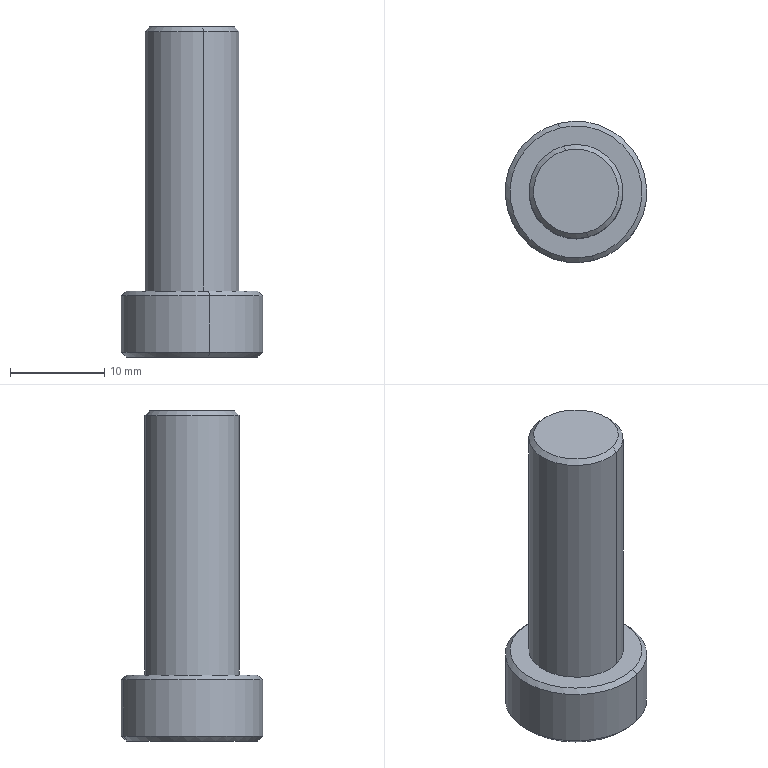Component | SolidWorks | JYTBJ-HeaderPlateBrakeAxis-1 | 1 solid | 17 faces | box 15 x 15 x 35 mm | volume 3077 mm3 | cone 8 | cylinder 6 | plane 3 | commonest cylinder face diameters 5 x2 10 x2 15 x2
build123d program:
from build123d import *

# Parameters (mm, degrees)
M6_TAPPED_HOLE1_D     = 5
M6_TAPPED_HOLE1_DEPTH = 17
M6_TAPPED_HOLE1_TIP   = 1.502
CHAMFER1_SIZE         = 0.5


with BuildPart() as part:
    # Sketch1 → Revolve1 (revolve)
    with BuildSketch(Plane.XY, mode=Mode.PRIVATE) as revolve1_sk:
        Polygon((0, 0), (7.5, 0), (7.5, 7), (5, 7), (5, 35), (0, 35), align=None)
    revolve(revolve1_sk.sketch.rotate(Axis((0, 0, 0), (0, 1, 0)), 90), axis=Axis((0, 0, 0), (0, 1, 0)))

    # M6 Tapped Hole1
    with Locations(Plane.XZ):
        with Locations((0, 0)):
            Hole(M6_TAPPED_HOLE1_D / 2, depth=M6_TAPPED_HOLE1_DEPTH)
            with Locations((0, 0, -(M6_TAPPED_HOLE1_DEPTH + M6_TAPPED_HOLE1_TIP / 2))):  # 118° drill point
                Cone(0, M6_TAPPED_HOLE1_D / 2, M6_TAPPED_HOLE1_TIP, mode=Mode.SUBTRACT)

    # Chamfer1
    chamfer1_edges = [part.edges().sort_by_distance(p)[0] for p in [
        (0, 35, 5),
        (0, 7, 7.5),
        (0, 0, 7.5),
    ]]
    chamfer(chamfer1_edges, length=CHAMFER1_SIZE)


solid = part.part

# Placed as in the assembly
solid = solid.moved(Location((35.724, 265.147, 18), (90, 0, 0)))
STEP:
#1=CARTESIAN_POINT('',(1.338,10.706,0.7087));
#2=VERTEX_POINT('',#1);
#3=CARTESIAN_POINT('',(1.475,10.172,0.7087));
#4=VERTEX_POINT('',#3);
#5=CARTESIAN_POINT('',(1.406,10.439,0.7087));
#6=DIRECTION('',(0.,0.,-1.));
#7=DIRECTION('',(-0.2502,0.9682,0.));
#8=AXIS2_PLACEMENT_3D('',#5,#6,#7);
#9=CIRCLE('',#8,0.2756);
#10=EDGE_CURVE('',#2,#4,#9,.T.);
#11=ORIENTED_EDGE('',*,*,#10,.F.);
#12=CARTESIAN_POINT('',(1.333,10.725,0.7283));
#13=VERTEX_POINT('',#12);
#14=CARTESIAN_POINT('',(1.338,10.706,0.7087));
#15=DIRECTION('',(-0.1769,0.6846,0.7071));
#16=VECTOR('',#15,39.37);
#17=LINE('',#14,#16);
#18=EDGE_CURVE('',#2,#13,#17,.T.);
#19=ORIENTED_EDGE('',*,*,#18,.T.);
#20=CARTESIAN_POINT('',(1.48,10.153,0.7283));
#21=VERTEX_POINT('',#20);
#22=CARTESIAN_POINT('',(1.406,10.439,0.7283));
#23=DIRECTION('',(0.,0.,1.));
#24=DIRECTION('',(-0.2502,0.9682,0.));
#25=AXIS2_PLACEMENT_3D('',#22,#23,#24);
#26=CIRCLE('',#25,0.2953);
#27=EDGE_CURVE('',#21,#13,#26,.T.);
#28=ORIENTED_EDGE('',*,*,#27,.F.);
#29=CARTESIAN_POINT('',(1.475,10.172,0.7087));
#30=DIRECTION('',(0.1769,-0.6846,0.7071));
#31=VECTOR('',#30,39.37);
#32=LINE('',#29,#31);
#33=EDGE_CURVE('',#4,#21,#32,.T.);
#34=ORIENTED_EDGE('',*,*,#33,.F.);
#35=EDGE_LOOP('',(#11,#19,#28,#34));
#36=FACE_OUTER_BOUND('',#35,.T.);
#37=CARTESIAN_POINT('',(1.406,10.439,0.7087));
#38=DIRECTION('',(0.,0.,1.));
#39=DIRECTION('',(0.2502,-0.9682,0.));
#40=AXIS2_PLACEMENT_3D('',#37,#38,#39);
#41=CONICAL_SURFACE('',#40,0.2756,0.7854);
#42=ADVANCED_FACE('',(#36),#41,.T.);
#43=CARTESIAN_POINT('',(1.475,10.172,0.9843));
#44=VERTEX_POINT('',#43);
#45=CARTESIAN_POINT('',(1.338,10.706,0.9843));
#46=VERTEX_POINT('',#45);
#47=CARTESIAN_POINT('',(1.406,10.439,0.9843));
#48=DIRECTION('',(0.,0.,1.));
#49=DIRECTION('',(0.2502,-0.9682,0.));
#50=AXIS2_PLACEMENT_3D('',#47,#48,#49);
#51=CIRCLE('',#50,0.2756);
#52=EDGE_CURVE('',#44,#46,#51,.T.);
#53=ORIENTED_EDGE('',*,*,#52,.F.);
#54=CARTESIAN_POINT('',(1.48,10.153,0.9646));
#55=VERTEX_POINT('',#54);
#56=CARTESIAN_POINT('',(1.48,10.153,0.9646));
#57=DIRECTION('',(0.1769,-0.6846,-0.7071));
#58=VECTOR('',#57,39.37);
#59=LINE('',#56,#58);
#60=EDGE_CURVE('',#44,#55,#59,.T.);
#61=ORIENTED_EDGE('',*,*,#60,.T.);
#62=CARTESIAN_POINT('',(1.333,10.725,0.9646));
#63=VERTEX_POINT('',#62);
#64=CARTESIAN_POINT('',(1.406,10.439,0.9646));
#65=DIRECTION('',(0.,0.,-1.));
#66=DIRECTION('',(0.2502,-0.9682,0.));
#67=AXIS2_PLACEMENT_3D('',#64,#65,#66);
#68=CIRCLE('',#67,0.2953);
#69=EDGE_CURVE('',#63,#55,#68,.T.);
#70=ORIENTED_EDGE('',*,*,#69,.F.);
#71=CARTESIAN_POINT('',(1.333,10.725,0.9646));
#72=DIRECTION('',(-0.1769,0.6846,-0.7071));
#73=VECTOR('',#72,39.37);
#74=LINE('',#71,#73);
#75=EDGE_CURVE('',#46,#63,#74,.T.);
#76=ORIENTED_EDGE('',*,*,#75,.F.);
#77=EDGE_LOOP('',(#53,#61,#70,#76));
#78=FACE_OUTER_BOUND('',#77,.T.);
#79=CARTESIAN_POINT('',(1.406,10.439,0.9646));
#80=DIRECTION('',(0.,0.,-1.));
#81=DIRECTION('',(-0.2502,0.9682,0.));
#82=AXIS2_PLACEMENT_3D('',#79,#80,#81);
#83=CONICAL_SURFACE('',#82,0.2953,0.7854);
#84=ADVANCED_FACE('',(#78),#83,.T.);
#85=CARTESIAN_POINT('',(1.451,10.267,2.087));
#86=VERTEX_POINT('',#85);
#87=CARTESIAN_POINT('',(1.362,10.61,2.087));
#88=VERTEX_POINT('',#87);
#89=CARTESIAN_POINT('',(1.406,10.439,2.087));
#90=DIRECTION('',(0.,0.,1.));
#91=DIRECTION('',(0.2502,-0.9682,0.));
#92=AXIS2_PLACEMENT_3D('',#89,#90,#91);
#93=CIRCLE('',#92,0.1772);
#94=EDGE_CURVE('',#86,#88,#93,.T.);
#95=ORIENTED_EDGE('',*,*,#94,.F.);
#96=CARTESIAN_POINT('',(1.456,10.248,2.067));
#97=VERTEX_POINT('',#96);
#98=CARTESIAN_POINT('',(1.456,10.248,2.067));
#99=DIRECTION('',(0.1769,-0.6846,-0.7071));
#100=VECTOR('',#99,39.37);
#101=LINE('',#98,#100);
#102=EDGE_CURVE('',#86,#97,#101,.T.);
#103=ORIENTED_EDGE('',*,*,#102,.T.);
#104=CARTESIAN_POINT('',(1.357,10.629,2.067));
#105=VERTEX_POINT('',#104);
#106=CARTESIAN_POINT('',(1.406,10.439,2.067));
#107=DIRECTION('',(0.,0.,-1.));
#108=DIRECTION('',(0.2502,-0.9682,0.));
#109=AXIS2_PLACEMENT_3D('',#106,#107,#108);
#110=CIRCLE('',#109,0.1969);
#111=EDGE_CURVE('',#105,#97,#110,.T.);
#112=ORIENTED_EDGE('',*,*,#111,.F.);
#113=CARTESIAN_POINT('',(1.357,10.629,2.067));
#114=DIRECTION('',(-0.1769,0.6846,-0.7071));
#115=VECTOR('',#114,39.37);
#116=LINE('',#113,#115);
#117=EDGE_CURVE('',#88,#105,#116,.T.);
#118=ORIENTED_EDGE('',*,*,#117,.F.);
#119=EDGE_LOOP('',(#95,#103,#112,#118));
#120=FACE_OUTER_BOUND('',#119,.T.);
#121=CARTESIAN_POINT('',(1.406,10.439,2.067));
#122=DIRECTION('',(0.,0.,-1.));
#123=DIRECTION('',(-0.2502,0.9682,0.));
#124=AXIS2_PLACEMENT_3D('',#121,#122,#123);
#125=CONICAL_SURFACE('',#124,0.1969,0.7854);
#126=ADVANCED_FACE('',(#120),#125,.T.);
#127=CARTESIAN_POINT('',(1.431,10.344,1.378));
#128=VERTEX_POINT('',#127);
#129=CARTESIAN_POINT('',(1.382,10.534,1.378));
#130=VERTEX_POINT('',#129);
#131=CARTESIAN_POINT('',(1.406,10.439,1.378));
#132=DIRECTION('',(0.,0.,-1.));
#133=DIRECTION('',(-0.2502,0.9682,0.));
#134=AXIS2_PLACEMENT_3D('',#131,#132,#133);
#135=CIRCLE('',#134,0.09843);
#136=EDGE_CURVE('',#128,#130,#135,.T.);
#137=ORIENTED_EDGE('',*,*,#136,.F.);
#138=CARTESIAN_POINT('',(1.431,10.344,0.7087));
#139=VERTEX_POINT('',#138);
#140=CARTESIAN_POINT('',(1.431,10.344,0.7087));
#141=DIRECTION('',(0.,0.,-1.));
#142=VECTOR('',#141,39.37);
#143=LINE('',#140,#142);
#144=EDGE_CURVE('',#128,#139,#143,.T.);
#145=ORIENTED_EDGE('',*,*,#144,.T.);
#146=CARTESIAN_POINT('',(1.382,10.534,0.7087));
#147=VERTEX_POINT('',#146);
#148=CARTESIAN_POINT('',(1.406,10.439,0.7087));
#149=DIRECTION('',(0.,0.,-1.));
#150=DIRECTION('',(-0.2502,0.9682,0.));
#151=AXIS2_PLACEMENT_3D('',#148,#149,#150);
#152=CIRCLE('',#151,0.09843);
#153=EDGE_CURVE('',#139,#147,#152,.T.);
#154=ORIENTED_EDGE('',*,*,#153,.T.);
#155=CARTESIAN_POINT('',(1.382,10.534,0.7087));
#156=DIRECTION('',(0.,0.,-1.));
#157=VECTOR('',#156,39.37);
#158=LINE('',#155,#157);
#159=EDGE_CURVE('',#130,#147,#158,.T.);
#160=ORIENTED_EDGE('',*,*,#159,.F.);
#161=EDGE_LOOP('',(#137,#145,#154,#160));
#162=FACE_OUTER_BOUND('',#161,.T.);
#163=CARTESIAN_POINT('',(1.406,10.439,0.7087));
#164=DIRECTION('',(0.,0.,-1.));
#165=DIRECTION('',(-0.2502,0.9682,0.));
#166=AXIS2_PLACEMENT_3D('',#163,#164,#165);
#167=CYLINDRICAL_SURFACE('',#166,0.09843);
#168=ADVANCED_FACE('',(#162),#167,.F.);
#169=CARTESIAN_POINT('',(1.406,10.439,1.437));
#170=VERTEX_POINT('',#169);
#171=CARTESIAN_POINT('',(1.382,10.534,1.378));
#172=DIRECTION('',(-0.2144,0.8299,-0.515));
#173=VECTOR('',#172,39.37);
#174=LINE('',#171,#173);
#175=EDGE_CURVE('',#170,#130,#174,.T.);
#176=ORIENTED_EDGE('',*,*,#175,.F.);
#177=CARTESIAN_POINT('',(1.431,10.344,1.378));
#178=DIRECTION('',(0.2144,-0.8299,-0.515));
#179=VECTOR('',#178,39.37);
#180=LINE('',#177,#179);
#181=EDGE_CURVE('',#170,#128,#180,.T.);
#182=ORIENTED_EDGE('',*,*,#181,.T.);
#183=ORIENTED_EDGE('',*,*,#136,.T.);
#184=EDGE_LOOP('',(#176,#182,#183));
#185=FACE_OUTER_BOUND('',#184,.T.);
#186=CARTESIAN_POINT('',(1.406,10.439,1.378));
#187=DIRECTION('',(0.,0.,-1.));
#188=DIRECTION('',(-0.2502,0.9682,0.));
#189=AXIS2_PLACEMENT_3D('',#186,#187,#188);
#190=CONICAL_SURFACE('',#189,0.09843,1.03);
#191=ADVANCED_FACE('',(#185),#190,.F.);
#192=ORIENTED_EDGE('',*,*,#111,.T.);
#193=CARTESIAN_POINT('',(1.456,10.248,0.9843));
#194=VERTEX_POINT('',#193);
#195=CARTESIAN_POINT('',(1.456,10.248,0.7087));
#196=DIRECTION('',(0.,0.,-1.));
#197=VECTOR('',#196,39.37);
#198=LINE('',#195,#197);
#199=EDGE_CURVE('',#97,#194,#198,.T.);
#200=ORIENTED_EDGE('',*,*,#199,.T.);
#201=CARTESIAN_POINT('',(1.357,10.629,0.9843));
#202=VERTEX_POINT('',#201);
#203=CARTESIAN_POINT('',(1.406,10.439,0.9843));
#204=DIRECTION('',(0.,0.,-1.));
#205=DIRECTION('',(-0.2502,0.9682,0.));
#206=AXIS2_PLACEMENT_3D('',#203,#204,#205);
#207=CIRCLE('',#206,0.1969);
#208=EDGE_CURVE('',#202,#194,#207,.T.);
#209=ORIENTED_EDGE('',*,*,#208,.F.);
#210=CARTESIAN_POINT('',(1.357,10.629,0.7087));
#211=DIRECTION('',(0.,0.,-1.));
#212=VECTOR('',#211,39.37);
#213=LINE('',#210,#212);
#214=EDGE_CURVE('',#105,#202,#213,.T.);
#215=ORIENTED_EDGE('',*,*,#214,.F.);
#216=EDGE_LOOP('',(#192,#200,#209,#215));
#217=FACE_OUTER_BOUND('',#216,.T.);
#218=CARTESIAN_POINT('',(1.406,10.439,0.7087));
#219=DIRECTION('',(0.,0.,-1.));
#220=DIRECTION('',(-0.2502,0.9682,0.));
#221=AXIS2_PLACEMENT_3D('',#218,#219,#220);
#222=CYLINDRICAL_SURFACE('',#221,0.1969);
#223=ADVANCED_FACE('',(#217),#222,.T.);
#224=ORIENTED_EDGE('',*,*,#69,.T.);
#225=CARTESIAN_POINT('',(1.48,10.153,0.7087));
#226=DIRECTION('',(0.,0.,-1.));
#227=VECTOR('',#226,39.37);
#228=LINE('',#225,#227);
#229=EDGE_CURVE('',#55,#21,#228,.T.);
#230=ORIENTED_EDGE('',*,*,#229,.T.);
#231=ORIENTED_EDGE('',*,*,#27,.T.);
#232=CARTESIAN_POINT('',(1.333,10.725,0.7087));
#233=DIRECTION('',(0.,0.,-1.));
#234=VECTOR('',#233,39.37);
#235=LINE('',#232,#234);
#236=EDGE_CURVE('',#63,#13,#235,.T.);
#237=ORIENTED_EDGE('',*,*,#236,.F.);
#238=EDGE_LOOP('',(#224,#230,#231,#237));
#239=FACE_OUTER_BOUND('',#238,.T.);
#240=CARTESIAN_POINT('',(1.406,10.439,0.7087));
#241=DIRECTION('',(0.,0.,-1.));
#242=DIRECTION('',(-0.2502,0.9682,0.));
#243=AXIS2_PLACEMENT_3D('',#240,#241,#242);
#244=CYLINDRICAL_SURFACE('',#243,0.2953);
#245=ADVANCED_FACE('',(#239),#244,.T.);
#246=CARTESIAN_POINT('',(1.406,10.439,0.7087));
#247=DIRECTION('',(0.,0.,-1.));
#248=DIRECTION('',(-0.2502,0.9682,0.));
#249=AXIS2_PLACEMENT_3D('',#246,#247,#248);
#250=CIRCLE('',#249,0.2756);
#251=EDGE_CURVE('',#4,#2,#250,.T.);
#252=ORIENTED_EDGE('',*,*,#251,.T.);
#253=ORIENTED_EDGE('',*,*,#10,.T.);
#254=EDGE_LOOP('',(#252,#253));
#255=FACE_OUTER_BOUND('',#254,.T.);
#256=CARTESIAN_POINT('',(1.406,10.439,0.7087));
#257=DIRECTION('',(0.,0.,-1.));
#258=DIRECTION('',(-0.2502,0.9682,0.));
#259=AXIS2_PLACEMENT_3D('',#256,#257,#258);
#260=CIRCLE('',#259,0.09843);
#261=EDGE_CURVE('',#147,#139,#260,.T.);
#262=ORIENTED_EDGE('',*,*,#261,.F.);
#263=ORIENTED_EDGE('',*,*,#153,.F.);
#264=EDGE_LOOP('',(#262,#263));
#265=FACE_BOUND('',#264,.T.);
#266=CARTESIAN_POINT('',(1.406,10.439,0.7087));
#267=DIRECTION('',(0.,0.,-1.));
#268=DIRECTION('',(-0.2502,0.9682,0.));
#269=AXIS2_PLACEMENT_3D('',#266,#267,#268);
#270=PLANE('',#269);
#271=ADVANCED_FACE('',(#255,#265),#270,.T.);
#272=ORIENTED_EDGE('',*,*,#229,.F.);
#273=CARTESIAN_POINT('',(1.406,10.439,0.9646));
#274=DIRECTION('',(0.,0.,-1.));
#275=DIRECTION('',(0.2502,-0.9682,0.));
#276=AXIS2_PLACEMENT_3D('',#273,#274,#275);
#277=CIRCLE('',#276,0.2953);
#278=EDGE_CURVE('',#55,#63,#277,.T.);
#279=ORIENTED_EDGE('',*,*,#278,.T.);
#280=ORIENTED_EDGE('',*,*,#236,.T.);
#281=CARTESIAN_POINT('',(1.406,10.439,0.7283));
#282=DIRECTION('',(0.,0.,1.));
#283=DIRECTION('',(-0.2502,0.9682,0.));
#284=AXIS2_PLACEMENT_3D('',#281,#282,#283);
#285=CIRCLE('',#284,0.2953);
#286=EDGE_CURVE('',#13,#21,#285,.T.);
#287=ORIENTED_EDGE('',*,*,#286,.T.);
#288=EDGE_LOOP('',(#272,#279,#280,#287));
#289=FACE_OUTER_BOUND('',#288,.T.);
#290=CARTESIAN_POINT('',(1.406,10.439,0.7087));
#291=DIRECTION('',(0.,0.,-1.));
#292=DIRECTION('',(-0.2502,0.9682,0.));
#293=AXIS2_PLACEMENT_3D('',#290,#291,#292);
#294=CYLINDRICAL_SURFACE('',#293,0.2953);
#295=ADVANCED_FACE('',(#289),#294,.T.);
#296=CARTESIAN_POINT('',(1.406,10.439,0.9843));
#297=DIRECTION('',(0.,0.,1.));
#298=DIRECTION('',(0.2502,-0.9682,0.));
#299=AXIS2_PLACEMENT_3D('',#296,#297,#298);
#300=CIRCLE('',#299,0.2756);
#301=EDGE_CURVE('',#46,#44,#300,.T.);
#302=ORIENTED_EDGE('',*,*,#301,.T.);
#303=ORIENTED_EDGE('',*,*,#52,.T.);
#304=EDGE_LOOP('',(#302,#303));
#305=FACE_OUTER_BOUND('',#304,.T.);
#306=ORIENTED_EDGE('',*,*,#208,.T.);
#307=CARTESIAN_POINT('',(1.406,10.439,0.9843));
#308=DIRECTION('',(0.,0.,-1.));
#309=DIRECTION('',(-0.2502,0.9682,0.));
#310=AXIS2_PLACEMENT_3D('',#307,#308,#309);
#311=CIRCLE('',#310,0.1969);
#312=EDGE_CURVE('',#194,#202,#311,.T.);
#313=ORIENTED_EDGE('',*,*,#312,.T.);
#314=EDGE_LOOP('',(#306,#313));
#315=FACE_BOUND('',#314,.T.);
#316=CARTESIAN_POINT('',(1.692,10.513,0.9843));
#317=DIRECTION('',(0.,0.,1.));
#318=DIRECTION('',(0.2502,-0.9682,0.));
#319=AXIS2_PLACEMENT_3D('',#316,#317,#318);
#320=PLANE('',#319);
#321=ADVANCED_FACE('',(#305,#315),#320,.T.);
#322=ORIENTED_EDGE('',*,*,#199,.F.);
#323=CARTESIAN_POINT('',(1.406,10.439,2.067));
#324=DIRECTION('',(0.,0.,-1.));
#325=DIRECTION('',(0.2502,-0.9682,0.));
#326=AXIS2_PLACEMENT_3D('',#323,#324,#325);
#327=CIRCLE('',#326,0.1969);
#328=EDGE_CURVE('',#97,#105,#327,.T.);
#329=ORIENTED_EDGE('',*,*,#328,.T.);
#330=ORIENTED_EDGE('',*,*,#214,.T.);
#331=ORIENTED_EDGE('',*,*,#312,.F.);
#332=EDGE_LOOP('',(#322,#329,#330,#331));
#333=FACE_OUTER_BOUND('',#332,.T.);
#334=CARTESIAN_POINT('',(1.406,10.439,0.7087));
#335=DIRECTION('',(0.,0.,-1.));
#336=DIRECTION('',(-0.2502,0.9682,0.));
#337=AXIS2_PLACEMENT_3D('',#334,#335,#336);
#338=CYLINDRICAL_SURFACE('',#337,0.1969);
#339=ADVANCED_FACE('',(#333),#338,.T.);
#340=CARTESIAN_POINT('',(1.406,10.439,2.087));
#341=DIRECTION('',(0.,0.,1.));
#342=DIRECTION('',(0.2502,-0.9682,0.));
#343=AXIS2_PLACEMENT_3D('',#340,#341,#342);
#344=CIRCLE('',#343,0.1772);
#345=EDGE_CURVE('',#88,#86,#344,.T.);
#346=ORIENTED_EDGE('',*,*,#345,.T.);
#347=ORIENTED_EDGE('',*,*,#94,.T.);
#348=EDGE_LOOP('',(#346,#347));
#349=FACE_OUTER_BOUND('',#348,.T.);
#350=CARTESIAN_POINT('',(1.597,10.488,2.087));
#351=DIRECTION('',(0.,0.,1.));
#352=DIRECTION('',(0.2502,-0.9682,0.));
#353=AXIS2_PLACEMENT_3D('',#350,#351,#352);
#354=PLANE('',#353);
#355=ADVANCED_FACE('',(#349),#354,.T.);
#356=ORIENTED_EDGE('',*,*,#181,.F.);
#357=ORIENTED_EDGE('',*,*,#175,.T.);
#358=CARTESIAN_POINT('',(1.406,10.439,1.378));
#359=DIRECTION('',(0.,0.,-1.));
#360=DIRECTION('',(-0.2502,0.9682,0.));
#361=AXIS2_PLACEMENT_3D('',#358,#359,#360);
#362=CIRCLE('',#361,0.09843);
#363=EDGE_CURVE('',#130,#128,#362,.T.);
#364=ORIENTED_EDGE('',*,*,#363,.T.);
#365=EDGE_LOOP('',(#356,#357,#364));
#366=FACE_OUTER_BOUND('',#365,.T.);
#367=CARTESIAN_POINT('',(1.406,10.439,1.378));
#368=DIRECTION('',(0.,0.,-1.));
#369=DIRECTION('',(-0.2502,0.9682,0.));
#370=AXIS2_PLACEMENT_3D('',#367,#368,#369);
#371=CONICAL_SURFACE('',#370,0.09843,1.03);
#372=ADVANCED_FACE('',(#366),#371,.F.);
#373=ORIENTED_EDGE('',*,*,#144,.F.);
#374=ORIENTED_EDGE('',*,*,#363,.F.);
#375=ORIENTED_EDGE('',*,*,#159,.T.);
#376=ORIENTED_EDGE('',*,*,#261,.T.);
#377=EDGE_LOOP('',(#373,#374,#375,#376));
#378=FACE_OUTER_BOUND('',#377,.T.);
#379=CARTESIAN_POINT('',(1.406,10.439,0.7087));
#380=DIRECTION('',(0.,0.,-1.));
#381=DIRECTION('',(-0.2502,0.9682,0.));
#382=AXIS2_PLACEMENT_3D('',#379,#380,#381);
#383=CYLINDRICAL_SURFACE('',#382,0.09843);
#384=ADVANCED_FACE('',(#378),#383,.F.);
#385=ORIENTED_EDGE('',*,*,#102,.F.);
#386=ORIENTED_EDGE('',*,*,#345,.F.);
#387=ORIENTED_EDGE('',*,*,#117,.T.);
#388=ORIENTED_EDGE('',*,*,#328,.F.);
#389=EDGE_LOOP('',(#385,#386,#387,#388));
#390=FACE_OUTER_BOUND('',#389,.T.);
#391=CARTESIAN_POINT('',(1.406,10.439,2.067));
#392=DIRECTION('',(0.,0.,-1.));
#393=DIRECTION('',(-0.2502,0.9682,0.));
#394=AXIS2_PLACEMENT_3D('',#391,#392,#393);
#395=CONICAL_SURFACE('',#394,0.1969,0.7854);
#396=ADVANCED_FACE('',(#390),#395,.T.);
#397=ORIENTED_EDGE('',*,*,#60,.F.);
#398=ORIENTED_EDGE('',*,*,#301,.F.);
#399=ORIENTED_EDGE('',*,*,#75,.T.);
#400=ORIENTED_EDGE('',*,*,#278,.F.);
#401=EDGE_LOOP('',(#397,#398,#399,#400));
#402=FACE_OUTER_BOUND('',#401,.T.);
#403=CARTESIAN_POINT('',(1.406,10.439,0.9646));
#404=DIRECTION('',(0.,0.,-1.));
#405=DIRECTION('',(-0.2502,0.9682,0.));
#406=AXIS2_PLACEMENT_3D('',#403,#404,#405);
#407=CONICAL_SURFACE('',#406,0.2953,0.7854);
#408=ADVANCED_FACE('',(#402),#407,.T.);
#409=ORIENTED_EDGE('',*,*,#18,.F.);
#410=ORIENTED_EDGE('',*,*,#251,.F.);
#411=ORIENTED_EDGE('',*,*,#33,.T.);
#412=ORIENTED_EDGE('',*,*,#286,.F.);
#413=EDGE_LOOP('',(#409,#410,#411,#412));
#414=FACE_OUTER_BOUND('',#413,.T.);
#415=CARTESIAN_POINT('',(1.406,10.439,0.7087));
#416=DIRECTION('',(0.,0.,1.));
#417=DIRECTION('',(0.2502,-0.9682,0.));
#418=AXIS2_PLACEMENT_3D('',#415,#416,#417);
#419=CONICAL_SURFACE('',#418,0.2756,0.7854);
#420=ADVANCED_FACE('',(#414),#419,.T.);
#421=CLOSED_SHELL('',(#42,#84,#126,#168,#191,#223,#245,#271,#295,#321,#339,#355,#372,#384,#396,#408,#420));
#422=MANIFOLD_SOLID_BREP('',#421);
#423=CARTESIAN_POINT('',(0.,0.,0.));
#424=DIRECTION('',(0.,0.,1.));
#425=DIRECTION('',(1.,0.,0.));
#426=AXIS2_PLACEMENT_3D('',#423,#424,#425);
#427=(LENGTH_UNIT()NAMED_UNIT(*)SI_UNIT($,.METRE.));
#428=LENGTH_MEASURE_WITH_UNIT(LENGTH_MEASURE(0.0254),#427);
#429=DIMENSIONAL_EXPONENTS(1.,0.,0.,0.,0.,0.,0.);
#430=(CONVERSION_BASED_UNIT('',#428)LENGTH_UNIT()NAMED_UNIT(#429));
#431=UNCERTAINTY_MEASURE_WITH_UNIT(LENGTH_MEASURE(0.00001),#430,'','');
#432=(NAMED_UNIT(*)PLANE_ANGLE_UNIT()SI_UNIT($,.RADIAN.));
#433=(NAMED_UNIT(*)SI_UNIT($,.STERADIAN.)SOLID_ANGLE_UNIT());
#434=(GEOMETRIC_REPRESENTATION_CONTEXT(3)GLOBAL_UNCERTAINTY_ASSIGNED_CONTEXT((#431))GLOBAL_UNIT_ASSIGNED_CONTEXT((#430,#432,#433))REPRESENTATION_CONTEXT('',''));
#435=ADVANCED_BREP_SHAPE_REPRESENTATION('',(#422,#426),#434);
#436=COLOUR_RGB('',0.7922,0.8196,0.9333);
#437=FILL_AREA_STYLE_COLOUR('',#436);
#438=FILL_AREA_STYLE('',(#437));
#439=SURFACE_STYLE_FILL_AREA(#438);
#440=SURFACE_SIDE_STYLE('',(#439));
#441=SURFACE_STYLE_USAGE(.BOTH.,#440);
#442=PRESENTATION_STYLE_ASSIGNMENT((#441));
#443=STYLED_ITEM('',(#442),#422);
#444=PRESENTATION_LAYER_ASSIGNMENT('','',(#443));
#445=(LENGTH_UNIT()NAMED_UNIT(*)SI_UNIT($,.METRE.));
#446=LENGTH_MEASURE_WITH_UNIT(LENGTH_MEASURE(0.0254),#445);
#447=DIMENSIONAL_EXPONENTS(1.,0.,0.,0.,0.,0.,0.);
#448=(CONVERSION_BASED_UNIT('',#446)LENGTH_UNIT()NAMED_UNIT(#447));
#449=UNCERTAINTY_MEASURE_WITH_UNIT(LENGTH_MEASURE(0.00001),#448,'','');
#450=(NAMED_UNIT(*)PLANE_ANGLE_UNIT()SI_UNIT($,.RADIAN.));
#451=(NAMED_UNIT(*)SI_UNIT($,.STERADIAN.)SOLID_ANGLE_UNIT());
#452=(GEOMETRIC_REPRESENTATION_CONTEXT(3)GLOBAL_UNCERTAINTY_ASSIGNED_CONTEXT((#449))GLOBAL_UNIT_ASSIGNED_CONTEXT((#448,#450,#451))REPRESENTATION_CONTEXT('',''));
#453=MECHANICAL_DESIGN_GEOMETRIC_PRESENTATION_REPRESENTATION('',(#443),#452);